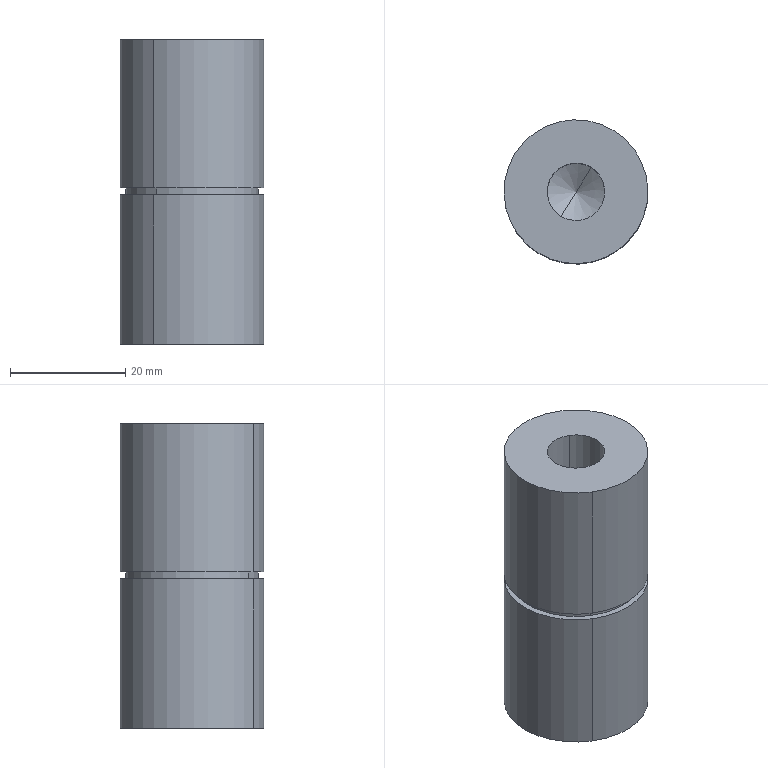Component | SolidWorks | SupportAxis-2 | 1 solid | 14 faces | box 25 x 25 x 53 mm | volume 22552 mm3 | cylinder 8 | plane 4 | cone 2 | commonest cylinder face diameters 25 x4 23 x2 10 x2
build123d program:
from build123d import *


with BuildPart() as part:
    # Sketch1 → Revolve1 (revolve)
    with BuildSketch(Plane.XY):
        Polygon((-11, 5), (-8.113, 0), (0, 0), (0, 12.5), (-26, 12.5), (-26, 11.5), (-27.2, 11.5), (-27.2, 12.5), (-53, 12.5), (-53, 5), align=None)
    revolve(axis=Axis((-53, 0, 0), (1, 0, 0)))


solid = part.part

# Placed as in the assembly
solid = solid.moved(Location((318, 551, -277.5), (0, 90, 0)))
STEP:
#1=COLOUR_RGB('',0.7922,0.8196,0.9333);
#2=FILL_AREA_STYLE_COLOUR('',#1);
#3=FILL_AREA_STYLE('',(#2));
#4=SURFACE_STYLE_FILL_AREA(#3);
#5=SURFACE_SIDE_STYLE('',(#4));
#6=SURFACE_STYLE_USAGE(.BOTH.,#5);
#7=PRESENTATION_STYLE_ASSIGNMENT((#6));
#8=CARTESIAN_POINT('',(12.78,22.11,-8.839));
#9=VERTEX_POINT('',#8);
#10=CARTESIAN_POINT('',(12.259,21.275,-8.839));
#11=VERTEX_POINT('',#10);
#12=CARTESIAN_POINT('',(12.52,21.693,-8.839));
#13=DIRECTION('',(-0.,-0.,-1.));
#14=DIRECTION('',(0.5294,0.8484,0.));
#15=AXIS2_PLACEMENT_3D('',#12,#13,#14);
#16=CIRCLE('',#15,0.4921);
#17=EDGE_CURVE('',#9,#11,#16,.T.);
#18=ORIENTED_EDGE('',*,*,#17,.T.);
#19=CARTESIAN_POINT('',(12.259,21.275,-9.854));
#20=VERTEX_POINT('',#19);
#21=CARTESIAN_POINT('',(12.259,21.275,-8.839));
#22=DIRECTION('',(-0.,-0.,-1.));
#23=VECTOR('',#22,39.37);
#24=LINE('',#21,#23);
#25=EDGE_CURVE('',#11,#20,#24,.T.);
#26=ORIENTED_EDGE('',*,*,#25,.T.);
#27=CARTESIAN_POINT('',(12.78,22.11,-9.854));
#28=VERTEX_POINT('',#27);
#29=CARTESIAN_POINT('',(12.52,21.693,-9.854));
#30=DIRECTION('',(-0.,-0.,-1.));
#31=DIRECTION('',(0.5294,0.8484,0.));
#32=AXIS2_PLACEMENT_3D('',#29,#30,#31);
#33=CIRCLE('',#32,0.4921);
#34=EDGE_CURVE('',#28,#20,#33,.T.);
#35=ORIENTED_EDGE('',*,*,#34,.F.);
#36=CARTESIAN_POINT('',(12.78,22.11,-8.839));
#37=DIRECTION('',(-0.,-0.,-1.));
#38=VECTOR('',#37,39.37);
#39=LINE('',#36,#38);
#40=EDGE_CURVE('',#9,#28,#39,.T.);
#41=ORIENTED_EDGE('',*,*,#40,.F.);
#42=EDGE_LOOP('',(#18,#26,#35,#41));
#43=FACE_OUTER_BOUND('',#42,.T.);
#44=CARTESIAN_POINT('',(12.52,21.693,-8.839));
#45=DIRECTION('',(-0.,-0.,-1.));
#46=DIRECTION('',(0.5294,0.8484,0.));
#47=AXIS2_PLACEMENT_3D('',#44,#45,#46);
#48=CYLINDRICAL_SURFACE('',#47,0.4921);
#49=ADVANCED_FACE('',(#43),#48,.T.);
#50=CARTESIAN_POINT('',(12.759,22.077,-9.854));
#51=VERTEX_POINT('',#50);
#52=CARTESIAN_POINT('',(12.28,21.309,-9.854));
#53=VERTEX_POINT('',#52);
#54=CARTESIAN_POINT('',(12.52,21.693,-9.854));
#55=DIRECTION('',(-0.,-0.,-1.));
#56=DIRECTION('',(0.5294,0.8484,0.));
#57=AXIS2_PLACEMENT_3D('',#54,#55,#56);
#58=CIRCLE('',#57,0.4528);
#59=EDGE_CURVE('',#51,#53,#58,.T.);
#60=ORIENTED_EDGE('',*,*,#59,.T.);
#61=CARTESIAN_POINT('',(12.28,21.309,-9.902));
#62=VERTEX_POINT('',#61);
#63=CARTESIAN_POINT('',(12.28,21.309,-8.839));
#64=DIRECTION('',(-0.,-0.,-1.));
#65=VECTOR('',#64,39.37);
#66=LINE('',#63,#65);
#67=EDGE_CURVE('',#53,#62,#66,.T.);
#68=ORIENTED_EDGE('',*,*,#67,.T.);
#69=CARTESIAN_POINT('',(12.759,22.077,-9.902));
#70=VERTEX_POINT('',#69);
#71=CARTESIAN_POINT('',(12.52,21.693,-9.902));
#72=DIRECTION('',(-0.,-0.,-1.));
#73=DIRECTION('',(0.5294,0.8484,0.));
#74=AXIS2_PLACEMENT_3D('',#71,#72,#73);
#75=CIRCLE('',#74,0.4528);
#76=EDGE_CURVE('',#70,#62,#75,.T.);
#77=ORIENTED_EDGE('',*,*,#76,.F.);
#78=CARTESIAN_POINT('',(12.759,22.077,-8.839));
#79=DIRECTION('',(-0.,-0.,-1.));
#80=VECTOR('',#79,39.37);
#81=LINE('',#78,#80);
#82=EDGE_CURVE('',#51,#70,#81,.T.);
#83=ORIENTED_EDGE('',*,*,#82,.F.);
#84=EDGE_LOOP('',(#60,#68,#77,#83));
#85=FACE_OUTER_BOUND('',#84,.T.);
#86=CARTESIAN_POINT('',(12.52,21.693,-8.839));
#87=DIRECTION('',(-0.,-0.,-1.));
#88=DIRECTION('',(0.5294,0.8484,0.));
#89=AXIS2_PLACEMENT_3D('',#86,#87,#88);
#90=CYLINDRICAL_SURFACE('',#89,0.4528);
#91=ADVANCED_FACE('',(#85),#90,.T.);
#92=CARTESIAN_POINT('',(12.78,22.11,-9.902));
#93=VERTEX_POINT('',#92);
#94=CARTESIAN_POINT('',(12.259,21.275,-9.902));
#95=VERTEX_POINT('',#94);
#96=CARTESIAN_POINT('',(12.52,21.693,-9.902));
#97=DIRECTION('',(-0.,-0.,-1.));
#98=DIRECTION('',(0.5294,0.8484,0.));
#99=AXIS2_PLACEMENT_3D('',#96,#97,#98);
#100=CIRCLE('',#99,0.4921);
#101=EDGE_CURVE('',#93,#95,#100,.T.);
#102=ORIENTED_EDGE('',*,*,#101,.T.);
#103=CARTESIAN_POINT('',(12.259,21.275,-10.925));
#104=VERTEX_POINT('',#103);
#105=CARTESIAN_POINT('',(12.259,21.275,-8.839));
#106=DIRECTION('',(-0.,-0.,-1.));
#107=VECTOR('',#106,39.37);
#108=LINE('',#105,#107);
#109=EDGE_CURVE('',#95,#104,#108,.T.);
#110=ORIENTED_EDGE('',*,*,#109,.T.);
#111=CARTESIAN_POINT('',(12.78,22.11,-10.925));
#112=VERTEX_POINT('',#111);
#113=CARTESIAN_POINT('',(12.52,21.693,-10.925));
#114=DIRECTION('',(-0.,-0.,-1.));
#115=DIRECTION('',(0.5294,0.8484,0.));
#116=AXIS2_PLACEMENT_3D('',#113,#114,#115);
#117=CIRCLE('',#116,0.4921);
#118=EDGE_CURVE('',#112,#104,#117,.T.);
#119=ORIENTED_EDGE('',*,*,#118,.F.);
#120=CARTESIAN_POINT('',(12.78,22.11,-8.839));
#121=DIRECTION('',(-0.,-0.,-1.));
#122=VECTOR('',#121,39.37);
#123=LINE('',#120,#122);
#124=EDGE_CURVE('',#93,#112,#123,.T.);
#125=ORIENTED_EDGE('',*,*,#124,.F.);
#126=EDGE_LOOP('',(#102,#110,#119,#125));
#127=FACE_OUTER_BOUND('',#126,.T.);
#128=CARTESIAN_POINT('',(12.52,21.693,-8.839));
#129=DIRECTION('',(-0.,-0.,-1.));
#130=DIRECTION('',(0.5294,0.8484,0.));
#131=AXIS2_PLACEMENT_3D('',#128,#129,#130);
#132=CYLINDRICAL_SURFACE('',#131,0.4921);
#133=ADVANCED_FACE('',(#127),#132,.T.);
#134=CARTESIAN_POINT('',(12.52,21.693,-10.606));
#135=VERTEX_POINT('',#134);
#136=CARTESIAN_POINT('',(12.415,21.526,-10.492));
#137=VERTEX_POINT('',#136);
#138=CARTESIAN_POINT('',(12.415,21.526,-10.492));
#139=DIRECTION('',(-0.4585,-0.7347,0.5));
#140=VECTOR('',#139,39.37);
#141=LINE('',#138,#140);
#142=EDGE_CURVE('',#135,#137,#141,.T.);
#143=ORIENTED_EDGE('',*,*,#142,.F.);
#144=CARTESIAN_POINT('',(12.624,21.86,-10.492));
#145=VERTEX_POINT('',#144);
#146=CARTESIAN_POINT('',(12.624,21.86,-10.492));
#147=DIRECTION('',(0.4585,0.7347,0.5));
#148=VECTOR('',#147,39.37);
#149=LINE('',#146,#148);
#150=EDGE_CURVE('',#135,#145,#149,.T.);
#151=ORIENTED_EDGE('',*,*,#150,.T.);
#152=CARTESIAN_POINT('',(12.52,21.693,-10.492));
#153=DIRECTION('',(-0.,-0.,-1.));
#154=DIRECTION('',(0.5294,0.8484,0.));
#155=AXIS2_PLACEMENT_3D('',#152,#153,#154);
#156=CIRCLE('',#155,0.1969);
#157=EDGE_CURVE('',#137,#145,#156,.T.);
#158=ORIENTED_EDGE('',*,*,#157,.F.);
#159=EDGE_LOOP('',(#143,#151,#158));
#160=FACE_OUTER_BOUND('',#159,.T.);
#161=CARTESIAN_POINT('',(12.52,21.693,-10.492));
#162=DIRECTION('',(0.,0.,1.));
#163=DIRECTION('',(-0.5294,-0.8484,0.));
#164=AXIS2_PLACEMENT_3D('',#161,#162,#163);
#165=CONICAL_SURFACE('',#164,0.1969,1.047);
#166=ADVANCED_FACE('',(#160),#165,.F.);
#167=CARTESIAN_POINT('',(12.415,21.526,-8.839));
#168=VERTEX_POINT('',#167);
#169=CARTESIAN_POINT('',(12.624,21.86,-8.839));
#170=VERTEX_POINT('',#169);
#171=CARTESIAN_POINT('',(12.52,21.693,-8.839));
#172=DIRECTION('',(-0.,-0.,-1.));
#173=DIRECTION('',(0.5294,0.8484,0.));
#174=AXIS2_PLACEMENT_3D('',#171,#172,#173);
#175=CIRCLE('',#174,0.1969);
#176=EDGE_CURVE('',#168,#170,#175,.T.);
#177=ORIENTED_EDGE('',*,*,#176,.F.);
#178=CARTESIAN_POINT('',(12.415,21.526,-8.839));
#179=DIRECTION('',(-0.,-0.,-1.));
#180=VECTOR('',#179,39.37);
#181=LINE('',#178,#180);
#182=EDGE_CURVE('',#168,#137,#181,.T.);
#183=ORIENTED_EDGE('',*,*,#182,.T.);
#184=ORIENTED_EDGE('',*,*,#157,.T.);
#185=CARTESIAN_POINT('',(12.624,21.86,-8.839));
#186=DIRECTION('',(-0.,-0.,-1.));
#187=VECTOR('',#186,39.37);
#188=LINE('',#185,#187);
#189=EDGE_CURVE('',#170,#145,#188,.T.);
#190=ORIENTED_EDGE('',*,*,#189,.F.);
#191=EDGE_LOOP('',(#177,#183,#184,#190));
#192=FACE_OUTER_BOUND('',#191,.T.);
#193=CARTESIAN_POINT('',(12.52,21.693,-8.839));
#194=DIRECTION('',(-0.,-0.,-1.));
#195=DIRECTION('',(0.5294,0.8484,0.));
#196=AXIS2_PLACEMENT_3D('',#193,#194,#195);
#197=CYLINDRICAL_SURFACE('',#196,0.1969);
#198=ADVANCED_FACE('',(#192),#197,.F.);
#199=ORIENTED_EDGE('',*,*,#182,.F.);
#200=CARTESIAN_POINT('',(12.52,21.693,-8.839));
#201=DIRECTION('',(-0.,-0.,-1.));
#202=DIRECTION('',(0.5294,0.8484,0.));
#203=AXIS2_PLACEMENT_3D('',#200,#201,#202);
#204=CIRCLE('',#203,0.1969);
#205=EDGE_CURVE('',#170,#168,#204,.T.);
#206=ORIENTED_EDGE('',*,*,#205,.F.);
#207=ORIENTED_EDGE('',*,*,#189,.T.);
#208=CARTESIAN_POINT('',(12.52,21.693,-10.492));
#209=DIRECTION('',(-0.,-0.,-1.));
#210=DIRECTION('',(0.5294,0.8484,0.));
#211=AXIS2_PLACEMENT_3D('',#208,#209,#210);
#212=CIRCLE('',#211,0.1969);
#213=EDGE_CURVE('',#145,#137,#212,.T.);
#214=ORIENTED_EDGE('',*,*,#213,.T.);
#215=EDGE_LOOP('',(#199,#206,#207,#214));
#216=FACE_OUTER_BOUND('',#215,.T.);
#217=CARTESIAN_POINT('',(12.52,21.693,-8.839));
#218=DIRECTION('',(-0.,-0.,-1.));
#219=DIRECTION('',(0.5294,0.8484,0.));
#220=AXIS2_PLACEMENT_3D('',#217,#218,#219);
#221=CYLINDRICAL_SURFACE('',#220,0.1969);
#222=ADVANCED_FACE('',(#216),#221,.F.);
#223=ORIENTED_EDGE('',*,*,#150,.F.);
#224=ORIENTED_EDGE('',*,*,#142,.T.);
#225=ORIENTED_EDGE('',*,*,#213,.F.);
#226=EDGE_LOOP('',(#223,#224,#225));
#227=FACE_OUTER_BOUND('',#226,.T.);
#228=CARTESIAN_POINT('',(12.52,21.693,-10.492));
#229=DIRECTION('',(0.,0.,1.));
#230=DIRECTION('',(-0.5294,-0.8484,0.));
#231=AXIS2_PLACEMENT_3D('',#228,#229,#230);
#232=CONICAL_SURFACE('',#231,0.1969,1.047);
#233=ADVANCED_FACE('',(#227),#232,.F.);
#234=ORIENTED_EDGE('',*,*,#118,.T.);
#235=CARTESIAN_POINT('',(12.52,21.693,-10.925));
#236=DIRECTION('',(-0.,-0.,-1.));
#237=DIRECTION('',(0.5294,0.8484,0.));
#238=AXIS2_PLACEMENT_3D('',#235,#236,#237);
#239=CIRCLE('',#238,0.4921);
#240=EDGE_CURVE('',#104,#112,#239,.T.);
#241=ORIENTED_EDGE('',*,*,#240,.T.);
#242=EDGE_LOOP('',(#234,#241));
#243=FACE_OUTER_BOUND('',#242,.T.);
#244=CARTESIAN_POINT('',(12.52,21.693,-10.925));
#245=DIRECTION('',(-0.,-0.,-1.));
#246=DIRECTION('',(0.5294,0.8484,-0.));
#247=AXIS2_PLACEMENT_3D('',#244,#245,#246);
#248=PLANE('',#247);
#249=ADVANCED_FACE('',(#243),#248,.T.);
#250=ORIENTED_EDGE('',*,*,#109,.F.);
#251=CARTESIAN_POINT('',(12.52,21.693,-9.902));
#252=DIRECTION('',(-0.,-0.,-1.));
#253=DIRECTION('',(0.5294,0.8484,0.));
#254=AXIS2_PLACEMENT_3D('',#251,#252,#253);
#255=CIRCLE('',#254,0.4921);
#256=EDGE_CURVE('',#95,#93,#255,.T.);
#257=ORIENTED_EDGE('',*,*,#256,.T.);
#258=ORIENTED_EDGE('',*,*,#124,.T.);
#259=ORIENTED_EDGE('',*,*,#240,.F.);
#260=EDGE_LOOP('',(#250,#257,#258,#259));
#261=FACE_OUTER_BOUND('',#260,.T.);
#262=CARTESIAN_POINT('',(12.52,21.693,-8.839));
#263=DIRECTION('',(-0.,-0.,-1.));
#264=DIRECTION('',(0.5294,0.8484,0.));
#265=AXIS2_PLACEMENT_3D('',#262,#263,#264);
#266=CYLINDRICAL_SURFACE('',#265,0.4921);
#267=ADVANCED_FACE('',(#261),#266,.T.);
#268=ORIENTED_EDGE('',*,*,#76,.T.);
#269=CARTESIAN_POINT('',(12.52,21.693,-9.902));
#270=DIRECTION('',(-0.,-0.,-1.));
#271=DIRECTION('',(0.5294,0.8484,0.));
#272=AXIS2_PLACEMENT_3D('',#269,#270,#271);
#273=CIRCLE('',#272,0.4528);
#274=EDGE_CURVE('',#62,#70,#273,.T.);
#275=ORIENTED_EDGE('',*,*,#274,.T.);
#276=EDGE_LOOP('',(#268,#275));
#277=FACE_BOUND('',#276,.T.);
#278=ORIENTED_EDGE('',*,*,#101,.F.);
#279=ORIENTED_EDGE('',*,*,#256,.F.);
#280=EDGE_LOOP('',(#278,#279));
#281=FACE_OUTER_BOUND('',#280,.T.);
#282=CARTESIAN_POINT('',(12.78,22.11,-9.902));
#283=DIRECTION('',(0.,0.,1.));
#284=DIRECTION('',(-0.5294,-0.8484,0.));
#285=AXIS2_PLACEMENT_3D('',#282,#283,#284);
#286=PLANE('',#285);
#287=ADVANCED_FACE('',(#277,#281),#286,.T.);
#288=ORIENTED_EDGE('',*,*,#67,.F.);
#289=CARTESIAN_POINT('',(12.52,21.693,-9.854));
#290=DIRECTION('',(-0.,-0.,-1.));
#291=DIRECTION('',(0.5294,0.8484,0.));
#292=AXIS2_PLACEMENT_3D('',#289,#290,#291);
#293=CIRCLE('',#292,0.4528);
#294=EDGE_CURVE('',#53,#51,#293,.T.);
#295=ORIENTED_EDGE('',*,*,#294,.T.);
#296=ORIENTED_EDGE('',*,*,#82,.T.);
#297=ORIENTED_EDGE('',*,*,#274,.F.);
#298=EDGE_LOOP('',(#288,#295,#296,#297));
#299=FACE_OUTER_BOUND('',#298,.T.);
#300=CARTESIAN_POINT('',(12.52,21.693,-8.839));
#301=DIRECTION('',(-0.,-0.,-1.));
#302=DIRECTION('',(0.5294,0.8484,0.));
#303=AXIS2_PLACEMENT_3D('',#300,#301,#302);
#304=CYLINDRICAL_SURFACE('',#303,0.4528);
#305=ADVANCED_FACE('',(#299),#304,.T.);
#306=ORIENTED_EDGE('',*,*,#34,.T.);
#307=CARTESIAN_POINT('',(12.52,21.693,-9.854));
#308=DIRECTION('',(-0.,-0.,-1.));
#309=DIRECTION('',(0.5294,0.8484,0.));
#310=AXIS2_PLACEMENT_3D('',#307,#308,#309);
#311=CIRCLE('',#310,0.4921);
#312=EDGE_CURVE('',#20,#28,#311,.T.);
#313=ORIENTED_EDGE('',*,*,#312,.T.);
#314=EDGE_LOOP('',(#306,#313));
#315=FACE_OUTER_BOUND('',#314,.T.);
#316=ORIENTED_EDGE('',*,*,#59,.F.);
#317=ORIENTED_EDGE('',*,*,#294,.F.);
#318=EDGE_LOOP('',(#316,#317));
#319=FACE_BOUND('',#318,.T.);
#320=CARTESIAN_POINT('',(12.759,22.077,-9.854));
#321=DIRECTION('',(-0.,-0.,-1.));
#322=DIRECTION('',(0.5294,0.8484,-0.));
#323=AXIS2_PLACEMENT_3D('',#320,#321,#322);
#324=PLANE('',#323);
#325=ADVANCED_FACE('',(#315,#319),#324,.T.);
#326=ORIENTED_EDGE('',*,*,#25,.F.);
#327=CARTESIAN_POINT('',(12.52,21.693,-8.839));
#328=DIRECTION('',(-0.,-0.,-1.));
#329=DIRECTION('',(0.5294,0.8484,0.));
#330=AXIS2_PLACEMENT_3D('',#327,#328,#329);
#331=CIRCLE('',#330,0.4921);
#332=EDGE_CURVE('',#11,#9,#331,.T.);
#333=ORIENTED_EDGE('',*,*,#332,.T.);
#334=ORIENTED_EDGE('',*,*,#40,.T.);
#335=ORIENTED_EDGE('',*,*,#312,.F.);
#336=EDGE_LOOP('',(#326,#333,#334,#335));
#337=FACE_OUTER_BOUND('',#336,.T.);
#338=CARTESIAN_POINT('',(12.52,21.693,-8.839));
#339=DIRECTION('',(-0.,-0.,-1.));
#340=DIRECTION('',(0.5294,0.8484,0.));
#341=AXIS2_PLACEMENT_3D('',#338,#339,#340);
#342=CYLINDRICAL_SURFACE('',#341,0.4921);
#343=ADVANCED_FACE('',(#337),#342,.T.);
#344=ORIENTED_EDGE('',*,*,#205,.T.);
#345=ORIENTED_EDGE('',*,*,#176,.T.);
#346=EDGE_LOOP('',(#344,#345));
#347=FACE_BOUND('',#346,.T.);
#348=ORIENTED_EDGE('',*,*,#17,.F.);
#349=ORIENTED_EDGE('',*,*,#332,.F.);
#350=EDGE_LOOP('',(#348,#349));
#351=FACE_OUTER_BOUND('',#350,.T.);
#352=CARTESIAN_POINT('',(12.78,22.11,-8.839));
#353=DIRECTION('',(0.,0.,1.));
#354=DIRECTION('',(-0.5294,-0.8484,0.));
#355=AXIS2_PLACEMENT_3D('',#352,#353,#354);
#356=PLANE('',#355);
#357=ADVANCED_FACE('',(#347,#351),#356,.T.);
#358=CLOSED_SHELL('',(#49,#91,#133,#166,#198,#222,#233,#249,#267,#287,#305,#325,#343,#357));
#359=MANIFOLD_SOLID_BREP('',#358);
#360=STYLED_ITEM('',(#7),#359);
#361=(LENGTH_UNIT()NAMED_UNIT(*)SI_UNIT($,.METRE.));
#362=LENGTH_MEASURE_WITH_UNIT(LENGTH_MEASURE(0.0254),#361);
#363=DIMENSIONAL_EXPONENTS(1.,0.,0.,0.,0.,0.,0.);
#364=(CONVERSION_BASED_UNIT('',#362)LENGTH_UNIT()NAMED_UNIT(#363));
#365=UNCERTAINTY_MEASURE_WITH_UNIT(LENGTH_MEASURE(0.00001),#364,'','');
#366=(NAMED_UNIT(*)PLANE_ANGLE_UNIT()SI_UNIT($,.RADIAN.));
#367=(NAMED_UNIT(*)SI_UNIT($,.STERADIAN.)SOLID_ANGLE_UNIT());
#368=(GEOMETRIC_REPRESENTATION_CONTEXT(3)GLOBAL_UNCERTAINTY_ASSIGNED_CONTEXT((#365))GLOBAL_UNIT_ASSIGNED_CONTEXT((#364,#366,#367))REPRESENTATION_CONTEXT('',''));
#369=MECHANICAL_DESIGN_GEOMETRIC_PRESENTATION_REPRESENTATION('',(#360),#368);
#370=CARTESIAN_POINT('',(0.,0.,0.));
#371=DIRECTION('',(0.,0.,1.));
#372=DIRECTION('',(1.,0.,0.));
#373=AXIS2_PLACEMENT_3D('',#370,#371,#372);
#374=(LENGTH_UNIT()NAMED_UNIT(*)SI_UNIT($,.METRE.));
#375=LENGTH_MEASURE_WITH_UNIT(LENGTH_MEASURE(0.0254),#374);
#376=DIMENSIONAL_EXPONENTS(1.,0.,0.,0.,0.,0.,0.);
#377=(CONVERSION_BASED_UNIT('',#375)LENGTH_UNIT()NAMED_UNIT(#376));
#378=UNCERTAINTY_MEASURE_WITH_UNIT(LENGTH_MEASURE(0.00001),#377,'','');
#379=(NAMED_UNIT(*)PLANE_ANGLE_UNIT()SI_UNIT($,.RADIAN.));
#380=(NAMED_UNIT(*)SI_UNIT($,.STERADIAN.)SOLID_ANGLE_UNIT());
#381=(GEOMETRIC_REPRESENTATION_CONTEXT(3)GLOBAL_UNCERTAINTY_ASSIGNED_CONTEXT((#378))GLOBAL_UNIT_ASSIGNED_CONTEXT((#377,#379,#380))REPRESENTATION_CONTEXT('',''));
#382=ADVANCED_BREP_SHAPE_REPRESENTATION('',(#359,#373),#381);
#383=PRESENTATION_LAYER_ASSIGNMENT('','',(#360));